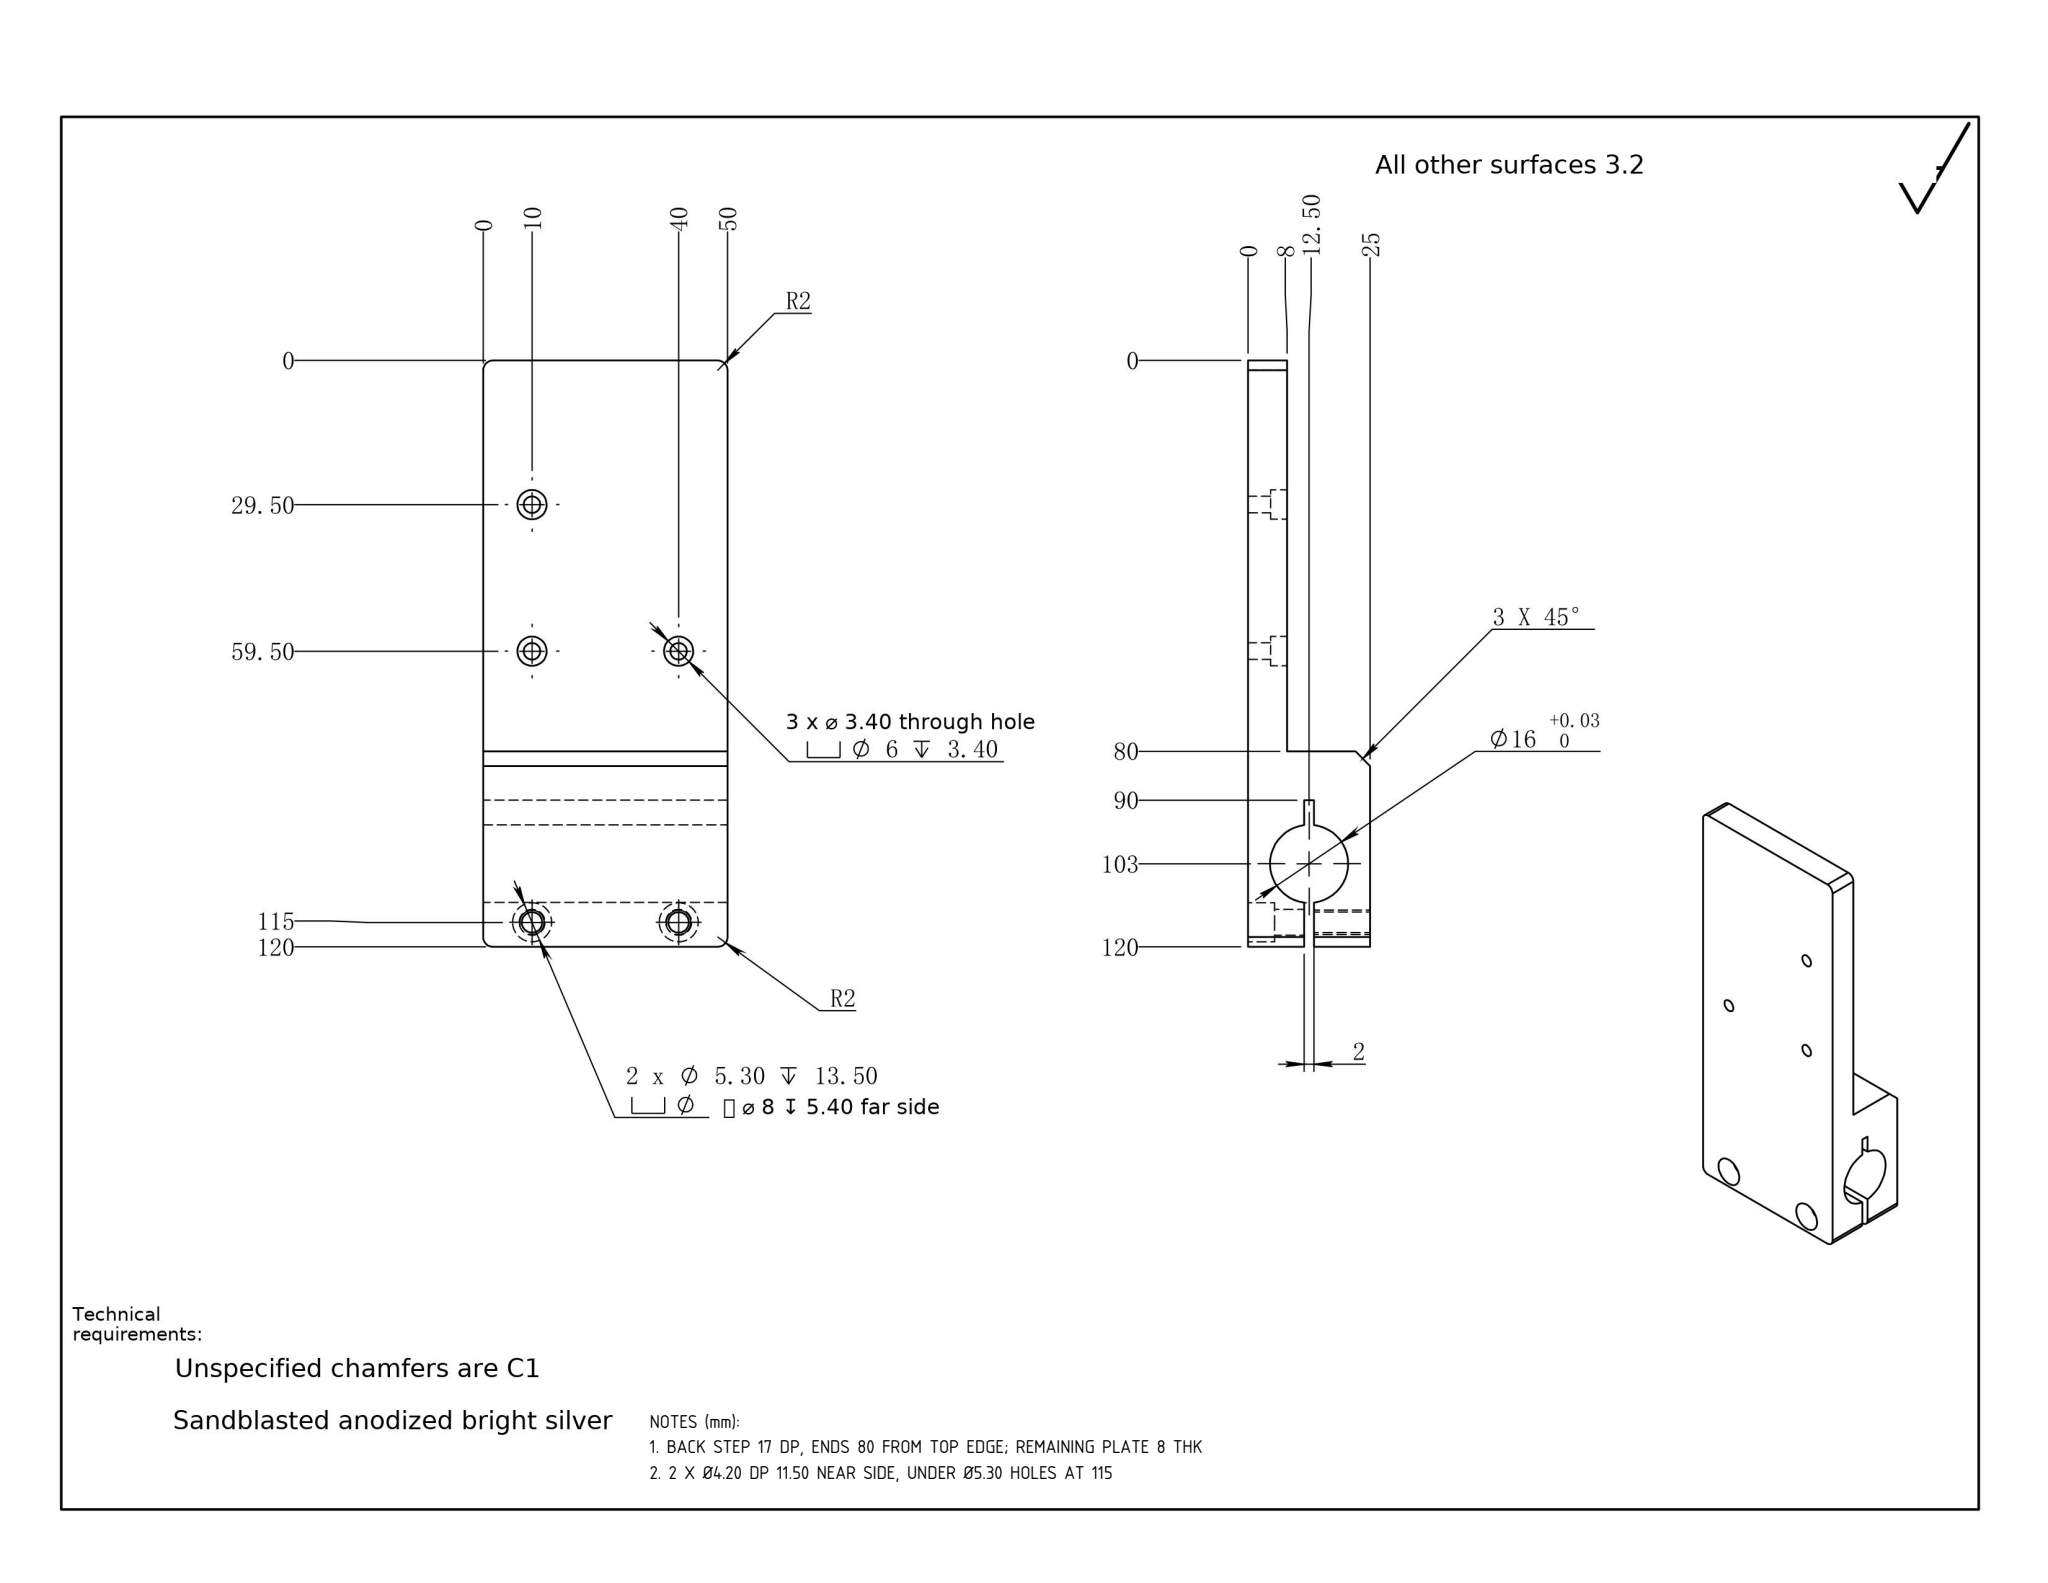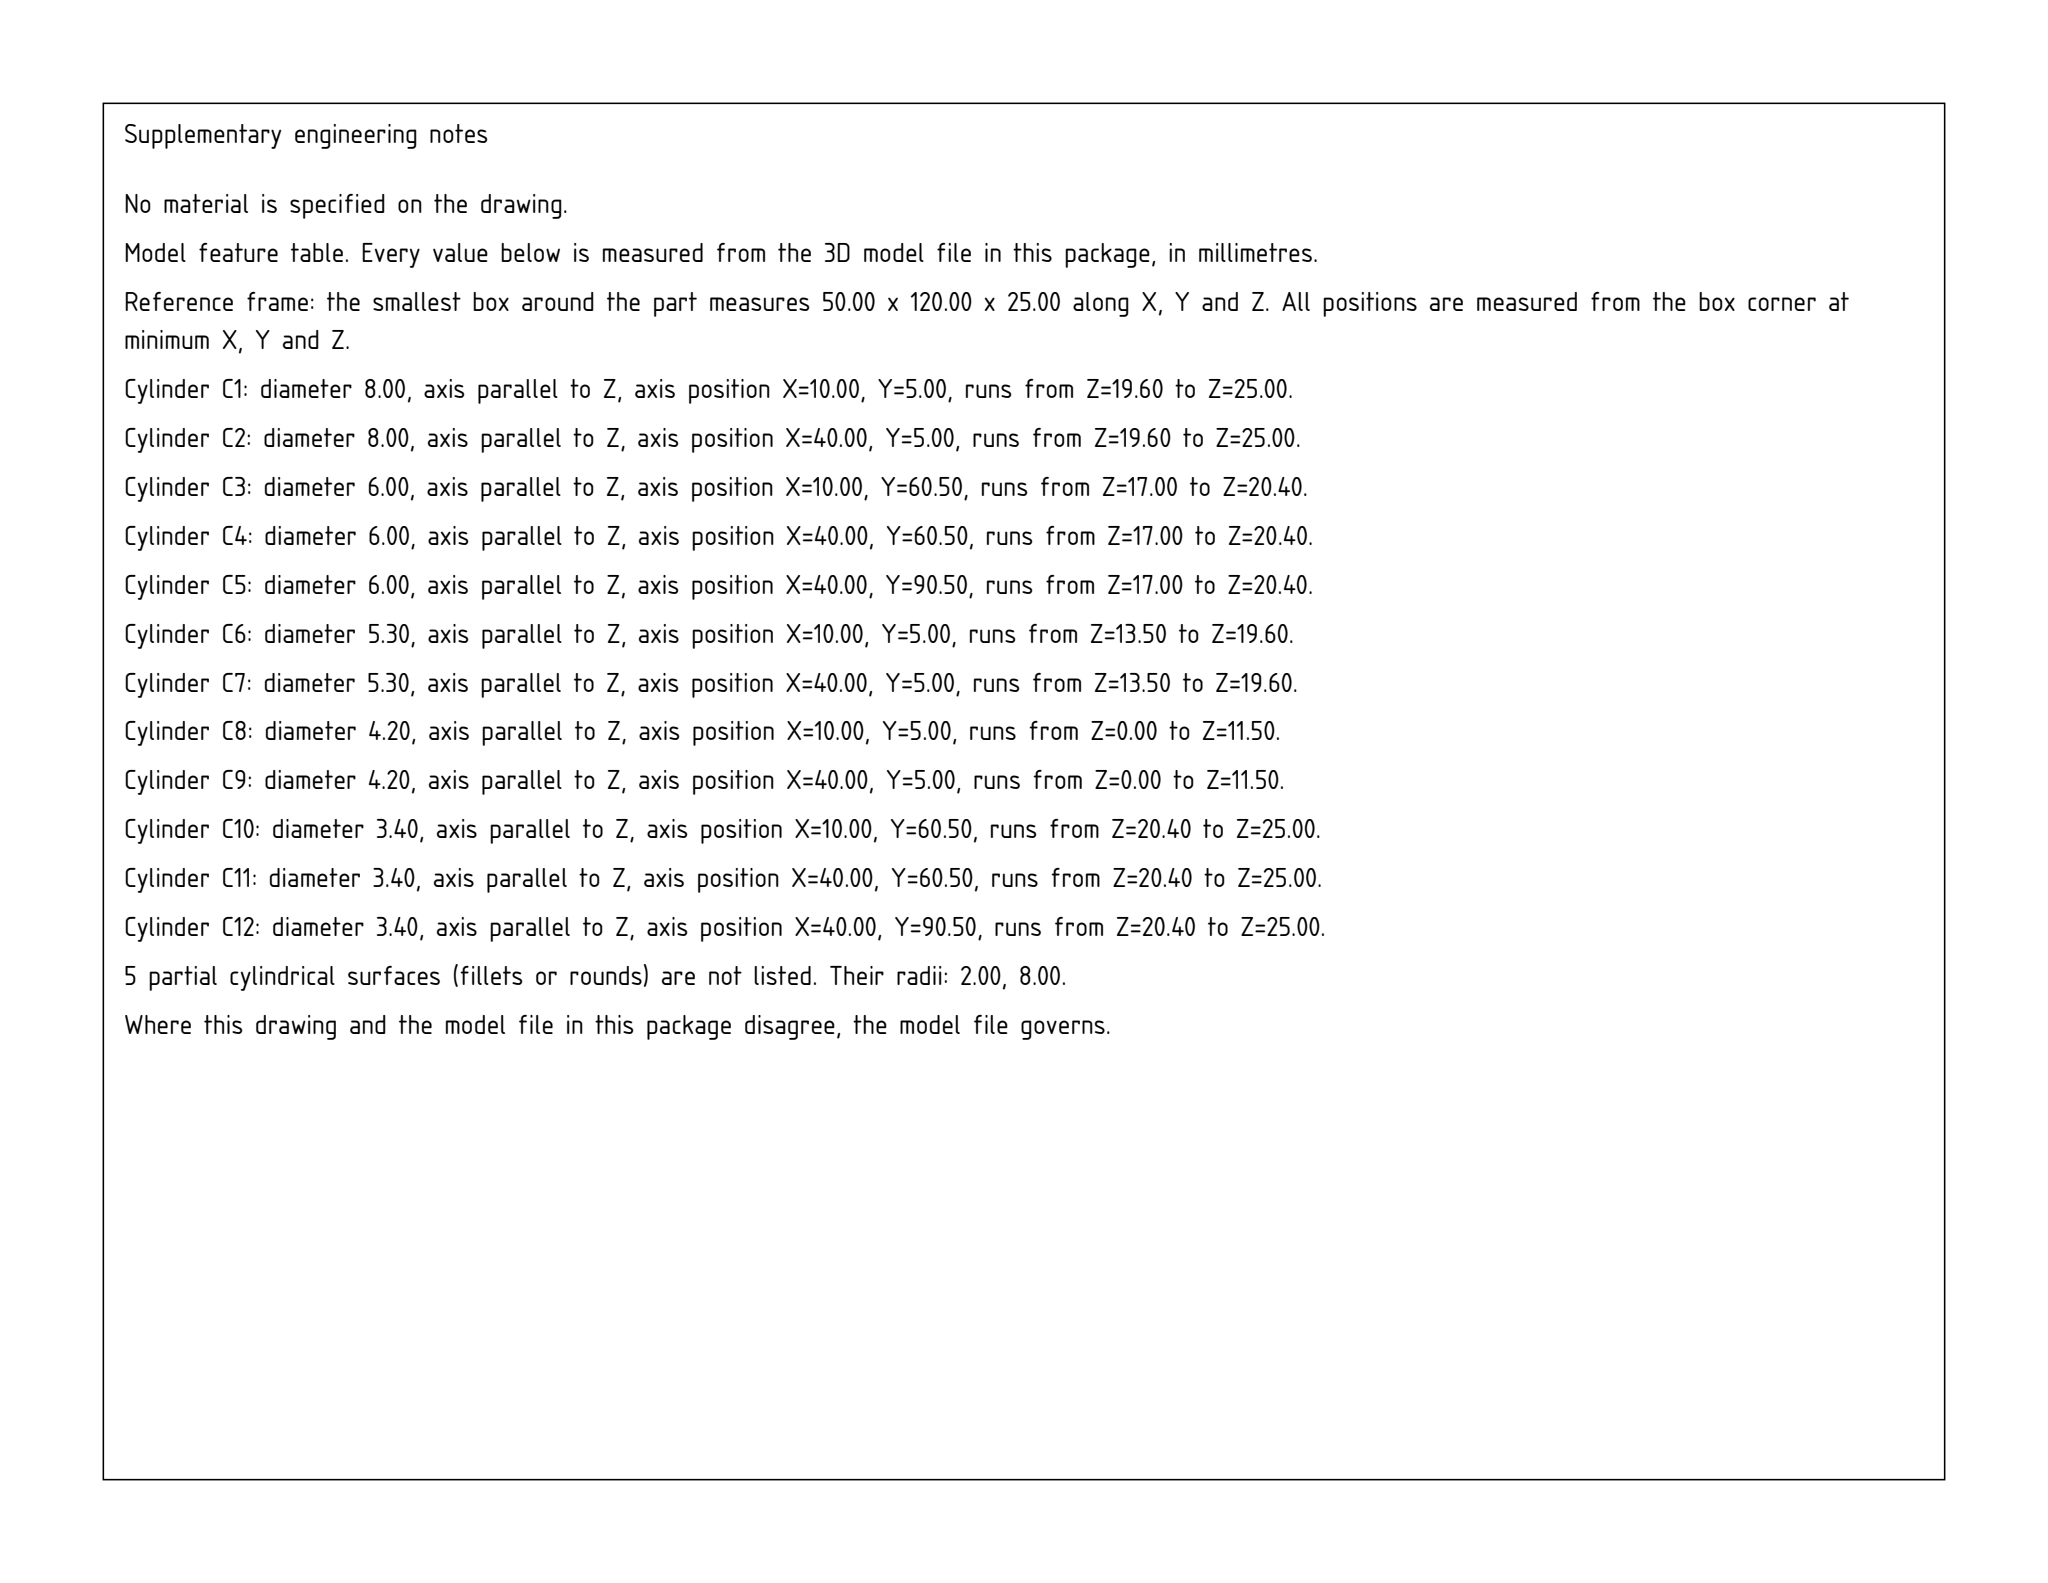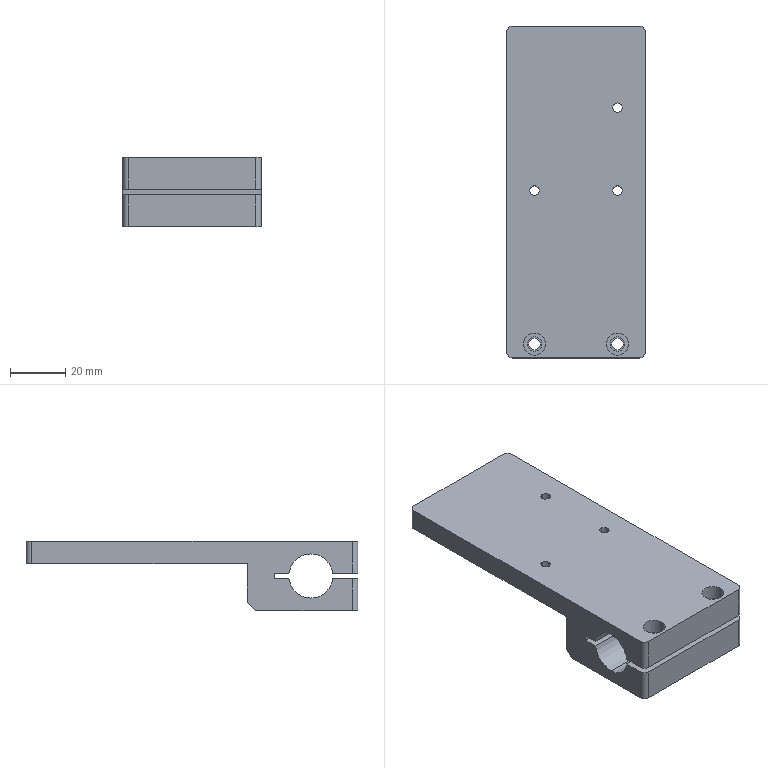Part | SolidWorks | mm | 1 solid | 53 faces | box 50 x 120 x 25 mm | volume 68720 mm3 | cylinder 33 | plane 20 | commonest cylinder face diameters 6 x6 3.4 x6 4 x6 8 x4 5.3 x4 4.2 x4 16 x3
Drawing notes:
BACK STEP 17 DP, ENDS 80 FROM TOP EDGE; REMAINING PLATE 8 THK | from the solid: z-planes 17.0 (step face) & 25.0 (back face) -> 25-17=8 thk; y-plane 40.0 = 80 from top edge y=120
2 X Ø4.20 DP 11.50 NEAR SIDE, UNDER Ø5.30 HOLES AT 115 | from the solid: Ø4.2 z-axis cyls at (10,5) & (40,5) len 11.5; Ø5.3 len 6.1 above them
build123d program:
from build123d import *

# Parameters (mm, degrees)
SKETCH1_W                                       = 50
SKETCH1_H                                       = 120
BOSS_EXTRUDE1_DEPTH                             = 12.5
SKETCH3_R                                       = 8
CUT_EXTRUDE1_DEPTH                              = 80.096
CUT_EXTRUDE2_DEPTH                              = 80.096
CUT_EXTRUDE2_DEPTH_BACK                         = 80.096
SKETCH4_W                                       = 2
SKETCH4_H                                       = 60
SKETCH5_W                                       = 17
SKETCH5_H                                       = 80
CUT_EXTRUDE3_DEPTH                              = 80.096
M3_HEX_SOCKET_HEAD_CAP_SCREW_CBORE1_D           = 3.4
M3_HEX_SOCKET_HEAD_CAP_SCREW_CBORE1_CBORE_D     = 6
M3_HEX_SOCKET_HEAD_CAP_SCREW_CBORE1_CBORE_DEPTH = 3.4
FILLET1_R                                       = 2
CHAMFER1_SIZE                                   = 3
M5_TAPPED_HOLE1_D                               = 4.2
M5_HEX_SOCKET_HEAD_CAP_SCREW_CBORE1_D           = 5.3
M5_HEX_SOCKET_HEAD_CAP_SCREW_CBORE1_DEPTH       = 13.499
M5_HEX_SOCKET_HEAD_CAP_SCREW_CBORE1_CBORE_D     = 8
M5_HEX_SOCKET_HEAD_CAP_SCREW_CBORE1_CBORE_DEPTH = 5.4


with BuildPart() as part:
    # Sketch1 → Boss-Extrude1 (new, symmetric)
    with BuildSketch(Plane.XY):
        Rectangle(SKETCH1_W, SKETCH1_H)
    extrude(amount=BOSS_EXTRUDE1_DEPTH, both=True)

    # Sketch3 → Cut-Extrude1 (cut, through all)
    with BuildSketch(Plane(origin=(25, 0, 0), x_dir=(0, 0, -1), z_dir=(1, 0, 0))):
        with Locations((0, -43)):
            Circle(SKETCH3_R)
    extrude(amount=-CUT_EXTRUDE1_DEPTH, mode=Mode.SUBTRACT)

    # Sketch4 → Cut-Extrude2 (cut, two sides: drawn at the far end of the back side and taken through both)
    with BuildSketch(Plane(origin=(25, 0, 0), x_dir=(0, 0, -1), z_dir=(1, 0, 0)).offset(-CUT_EXTRUDE2_DEPTH_BACK)):
        with Locations((0, -60)):
            Rectangle(SKETCH4_W, SKETCH4_H)
    extrude(amount=CUT_EXTRUDE2_DEPTH + CUT_EXTRUDE2_DEPTH_BACK, mode=Mode.SUBTRACT)

    # Sketch5 → Cut-Extrude3 (cut, through all)
    with BuildSketch(Plane(origin=(25, 0, 0), x_dir=(0, 0, -1), z_dir=(1, 0, 0))):
        with Locations((4, 20)):
            Rectangle(SKETCH5_W, SKETCH5_H)
    extrude(amount=-CUT_EXTRUDE3_DEPTH, mode=Mode.SUBTRACT)

    # M3 Hex Socket Head Cap Screw CBORE1 (through all)
    with Locations(Plane(origin=(0, 0, 4.5), x_dir=(-1, 0, 0), z_dir=(0, 0, -1))):
        with Locations((-15, 30.5), (15, 0.5), (-15, 0.5)):
            CounterBoreHole(M3_HEX_SOCKET_HEAD_CAP_SCREW_CBORE1_D / 2, M3_HEX_SOCKET_HEAD_CAP_SCREW_CBORE1_CBORE_D / 2, M3_HEX_SOCKET_HEAD_CAP_SCREW_CBORE1_CBORE_DEPTH)

    # Fillet1
    fillet1_edges = [part.edges().sort_by_distance(p)[0] for p in [
        (25, -60, -6.75),
        (-25, -60, -6.75),
        (25, -60, 6.75),
        (-25, -60, 6.75),
        (-25, 60, 8.5),
        (25, 60, 8.5),
    ]]
    fillet(fillet1_edges, radius=FILLET1_R)

    # Chamfer1
    chamfer1_edges = [part.edges().sort_by_distance(p)[0] for p in [
        (0, -20, -12.5),
    ]]
    chamfer(chamfer1_edges, length=CHAMFER1_SIZE)

    # M5 Tapped Hole1 (through all)
    with Locations(Plane(origin=(0, 0, -12.5), x_dir=(-1, 0, 0), z_dir=(0, 0, -1))):
        with Locations((15, -55), (-15, -55)):
            Hole(M5_TAPPED_HOLE1_D / 2)

    # M5 Hex Socket Head Cap Screw CBORE1
    with Locations(Plane(origin=(0, 0, 12.5), x_dir=(-1, 0, 0), z_dir=(0, 0, 1))):
        with Locations((-15, 55), (15, 55)):
            CounterBoreHole(M5_HEX_SOCKET_HEAD_CAP_SCREW_CBORE1_D / 2, M5_HEX_SOCKET_HEAD_CAP_SCREW_CBORE1_CBORE_D / 2, M5_HEX_SOCKET_HEAD_CAP_SCREW_CBORE1_CBORE_DEPTH, depth=M5_HEX_SOCKET_HEAD_CAP_SCREW_CBORE1_DEPTH)


solid = part.part